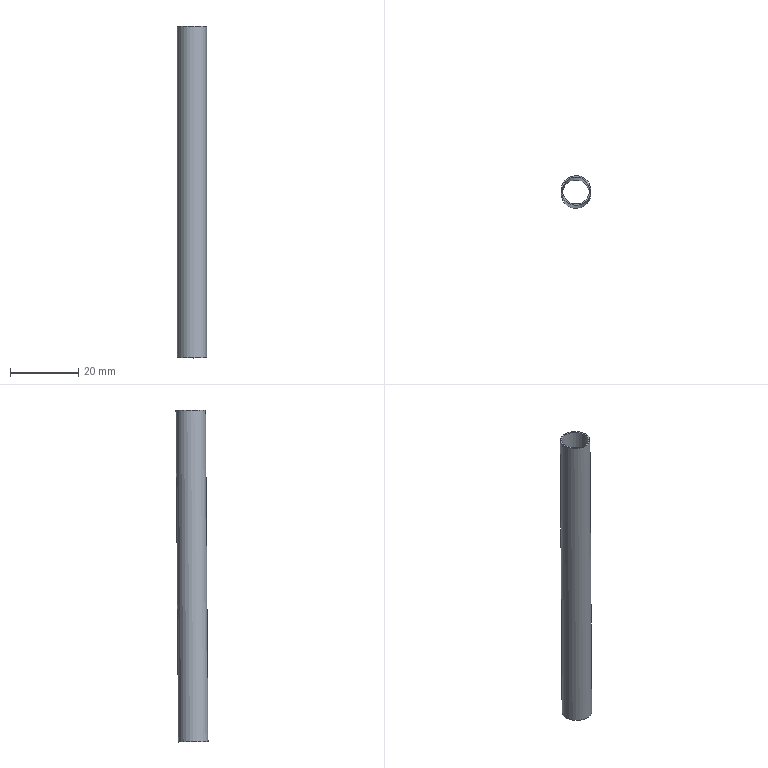Component | NX | TUBE_1 | 1 solid | 4 faces | box 8.7 x 9.44 x 97.29 mm | volume 1014 mm3 | plane 2 | cylinder 2 | commonest cylinder face diameters 8.7 x1 7.9 x1
STEP:
#1=CARTESIAN_POINT('',(0.,0.,0.));
#2=DIRECTION('',(0.,0.,1.));
#3=DIRECTION('',(1.,0.,0.));
#4=AXIS2_PLACEMENT_3D('',#1,#2,#3);
#5=CARTESIAN_POINT('',(51.171,-45.272,126.869));
#6=VERTEX_POINT('',#5);
#7=CARTESIAN_POINT('',(47.221,-45.312,126.87));
#8=DIRECTION('',(-0.0000015,-0.007573,-1.));
#9=DIRECTION('',(0.9999,0.01011,-0.00007807));
#10=AXIS2_PLACEMENT_3D('',#7,#8,#9);
#11=CIRCLE('',#10,3.95);
#12=CARTESIAN_POINT('',(47.221,-45.312,126.87));
#13=DIRECTION('',(0.0000015,0.007573,1.));
#14=DIRECTION('',(0.9999,0.01011,-0.00007807));
#15=AXIS2_PLACEMENT_3D('',#12,#13,#14);
#16=PLANE('',#15);
#17=CARTESIAN_POINT('',(3.95,0.));
#18=CARTESIAN_POINT('',(3.95,-6.842));
#19=CARTESIAN_POINT('',(-1.975,-3.421));
#20=CARTESIAN_POINT('',(-7.9,-0.));
#21=CARTESIAN_POINT('',(-1.975,3.421));
#22=CARTESIAN_POINT('',(3.95,6.842));
#23=CARTESIAN_POINT('',(3.95,0.));
#24=(BOUNDED_CURVE()B_SPLINE_CURVE(2,(#17,#18,#19,#20,#21,#22,#23),.UNSPECIFIED.,.T.,.F.)B_SPLINE_CURVE_WITH_KNOTS((1,2,2,2,2,1),(-2.094,0.,2.094,4.189,6.283,8.378),.UNSPECIFIED.)CURVE()GEOMETRIC_REPRESENTATION_ITEM()RATIONAL_B_SPLINE_CURVE((1.,0.5,1.,0.5,1.,0.5,1.))REPRESENTATION_ITEM(''));
#25=(GEOMETRIC_REPRESENTATION_CONTEXT(2)PARAMETRIC_REPRESENTATION_CONTEXT()REPRESENTATION_CONTEXT('',''));
#26=DEFINITIONAL_REPRESENTATION('',(#24),#25);
#27=PCURVE('',#16,#26);
#28=CARTESIAN_POINT('',(47.221,-46.048,29.642));
#29=DIRECTION('',(0.0000015,0.007573,1.));
#30=DIRECTION('',(0.9999,0.01011,-0.00007807));
#31=AXIS2_PLACEMENT_3D('',#28,#29,#30);
#32=CYLINDRICAL_SURFACE('',#31,3.95);
#33=CARTESIAN_POINT('',(6.283,97.23));
#34=DIRECTION('',(-1.,0.));
#35=VECTOR('',#34,1.);
#36=LINE('',#33,#35);
#37=(GEOMETRIC_REPRESENTATION_CONTEXT(2)PARAMETRIC_REPRESENTATION_CONTEXT()REPRESENTATION_CONTEXT('',''));
#38=DEFINITIONAL_REPRESENTATION('',(#36),#37);
#39=PCURVE('',#32,#38);
#40=SURFACE_CURVE('',#11,(#27,#39),.PCURVE_S1.);
#41=EDGE_CURVE('',#6,#6,#40,.T.);
#42=ORIENTED_EDGE('',*,*,#41,.T.);
#43=EDGE_LOOP('',(#42));
#44=FACE_BOUND('',#43,.T.);
#45=CARTESIAN_POINT('',(51.571,-45.268,126.869));
#46=VERTEX_POINT('',#45);
#47=CARTESIAN_POINT('',(47.221,-45.312,126.87));
#48=DIRECTION('',(-0.0000015,-0.007573,-1.));
#49=DIRECTION('',(0.9999,0.01011,-0.00007807));
#50=AXIS2_PLACEMENT_3D('',#47,#48,#49);
#51=CIRCLE('',#50,4.35);
#52=CARTESIAN_POINT('',(4.35,0.));
#53=CARTESIAN_POINT('',(4.35,-7.534));
#54=CARTESIAN_POINT('',(-2.175,-3.767));
#55=CARTESIAN_POINT('',(-8.7,-0.));
#56=CARTESIAN_POINT('',(-2.175,3.767));
#57=CARTESIAN_POINT('',(4.35,7.534));
#58=CARTESIAN_POINT('',(4.35,0.));
#59=(BOUNDED_CURVE()B_SPLINE_CURVE(2,(#52,#53,#54,#55,#56,#57,#58),.UNSPECIFIED.,.T.,.F.)B_SPLINE_CURVE_WITH_KNOTS((1,2,2,2,2,1),(-2.094,0.,2.094,4.189,6.283,8.378),.UNSPECIFIED.)CURVE()GEOMETRIC_REPRESENTATION_ITEM()RATIONAL_B_SPLINE_CURVE((1.,0.5,1.,0.5,1.,0.5,1.))REPRESENTATION_ITEM(''));
#60=(GEOMETRIC_REPRESENTATION_CONTEXT(2)PARAMETRIC_REPRESENTATION_CONTEXT()REPRESENTATION_CONTEXT('',''));
#61=DEFINITIONAL_REPRESENTATION('',(#59),#60);
#62=PCURVE('',#16,#61);
#63=CARTESIAN_POINT('',(47.221,-46.048,29.642));
#64=DIRECTION('',(0.0000015,0.007573,1.));
#65=DIRECTION('',(0.9999,0.01011,-0.00007807));
#66=AXIS2_PLACEMENT_3D('',#63,#64,#65);
#67=CYLINDRICAL_SURFACE('',#66,4.35);
#68=CARTESIAN_POINT('',(6.283,97.23));
#69=DIRECTION('',(-1.,0.));
#70=VECTOR('',#69,1.);
#71=LINE('',#68,#70);
#72=(GEOMETRIC_REPRESENTATION_CONTEXT(2)PARAMETRIC_REPRESENTATION_CONTEXT()REPRESENTATION_CONTEXT('',''));
#73=DEFINITIONAL_REPRESENTATION('',(#71),#72);
#74=PCURVE('',#67,#73);
#75=SURFACE_CURVE('',#51,(#62,#74),.PCURVE_S1.);
#76=EDGE_CURVE('',#46,#46,#75,.T.);
#77=ORIENTED_EDGE('',*,*,#76,.F.);
#78=EDGE_LOOP('',(#77));
#79=FACE_BOUND('',#78,.T.);
#80=ADVANCED_FACE('',(#44,#79),#16,.T.);
#81=CARTESIAN_POINT('',(43.271,-46.088,29.643));
#82=VERTEX_POINT('',#81);
#83=CARTESIAN_POINT('',(51.171,-46.008,29.642));
#84=VERTEX_POINT('',#83);
#85=CARTESIAN_POINT('',(47.221,-46.048,29.642));
#86=DIRECTION('',(0.0000015,0.007573,1.));
#87=DIRECTION('',(-0.9999,-0.01011,0.00007807));
#88=AXIS2_PLACEMENT_3D('',#85,#86,#87);
#89=CIRCLE('',#88,3.95);
#90=CARTESIAN_POINT('',(47.221,-46.048,29.642));
#91=DIRECTION('',(-0.0000015,-0.007573,-1.));
#92=DIRECTION('',(-0.9999,-0.01011,0.00007807));
#93=AXIS2_PLACEMENT_3D('',#90,#91,#92);
#94=PLANE('',#93);
#95=CARTESIAN_POINT('',(3.95,-0.));
#96=CARTESIAN_POINT('',(3.95,-6.842));
#97=CARTESIAN_POINT('',(-1.975,-3.421));
#98=CARTESIAN_POINT('',(-7.9,0.));
#99=CARTESIAN_POINT('',(-1.975,3.421));
#100=CARTESIAN_POINT('',(3.95,6.842));
#101=CARTESIAN_POINT('',(3.95,-0.));
#102=(BOUNDED_CURVE()B_SPLINE_CURVE(2,(#95,#96,#97,#98,#99,#100,#101),.UNSPECIFIED.,.T.,.F.)B_SPLINE_CURVE_WITH_KNOTS((1,2,2,2,2,1),(-2.094,0.,2.094,4.189,6.283,8.378),.UNSPECIFIED.)CURVE()GEOMETRIC_REPRESENTATION_ITEM()RATIONAL_B_SPLINE_CURVE((1.,0.5,1.,0.5,1.,0.5,1.))REPRESENTATION_ITEM(''));
#103=(GEOMETRIC_REPRESENTATION_CONTEXT(2)PARAMETRIC_REPRESENTATION_CONTEXT()REPRESENTATION_CONTEXT('',''));
#104=DEFINITIONAL_REPRESENTATION('',(#102),#103);
#105=PCURVE('',#94,#104);
#106=CARTESIAN_POINT('',(3.142,0.));
#107=DIRECTION('',(1.,0.));
#108=VECTOR('',#107,1.);
#109=LINE('',#106,#108);
#110=(GEOMETRIC_REPRESENTATION_CONTEXT(2)PARAMETRIC_REPRESENTATION_CONTEXT()REPRESENTATION_CONTEXT('',''));
#111=DEFINITIONAL_REPRESENTATION('',(#109),#110);
#112=PCURVE('',#32,#111);
#113=SURFACE_CURVE('',#89,(#105,#112),.PCURVE_S1.);
#114=EDGE_CURVE('',#82,#84,#113,.T.);
#115=ORIENTED_EDGE('',*,*,#114,.T.);
#116=CARTESIAN_POINT('',(47.221,-46.048,29.642));
#117=DIRECTION('',(0.0000015,0.007573,1.));
#118=DIRECTION('',(-0.9999,-0.01011,0.00007807));
#119=AXIS2_PLACEMENT_3D('',#116,#117,#118);
#120=CIRCLE('',#119,3.95);
#121=CARTESIAN_POINT('',(3.95,-0.));
#122=CARTESIAN_POINT('',(3.95,-6.842));
#123=CARTESIAN_POINT('',(-1.975,-3.421));
#124=CARTESIAN_POINT('',(-7.9,0.));
#125=CARTESIAN_POINT('',(-1.975,3.421));
#126=CARTESIAN_POINT('',(3.95,6.842));
#127=CARTESIAN_POINT('',(3.95,-0.));
#128=(BOUNDED_CURVE()B_SPLINE_CURVE(2,(#121,#122,#123,#124,#125,#126,#127),.UNSPECIFIED.,.T.,.F.)B_SPLINE_CURVE_WITH_KNOTS((1,2,2,2,2,1),(-2.094,0.,2.094,4.189,6.283,8.378),.UNSPECIFIED.)CURVE()GEOMETRIC_REPRESENTATION_ITEM()RATIONAL_B_SPLINE_CURVE((1.,0.5,1.,0.5,1.,0.5,1.))REPRESENTATION_ITEM(''));
#129=(GEOMETRIC_REPRESENTATION_CONTEXT(2)PARAMETRIC_REPRESENTATION_CONTEXT()REPRESENTATION_CONTEXT('',''));
#130=DEFINITIONAL_REPRESENTATION('',(#128),#129);
#131=PCURVE('',#94,#130);
#132=CARTESIAN_POINT('',(-3.142,0.));
#133=DIRECTION('',(1.,0.));
#134=VECTOR('',#133,1.);
#135=LINE('',#132,#134);
#136=(GEOMETRIC_REPRESENTATION_CONTEXT(2)PARAMETRIC_REPRESENTATION_CONTEXT()REPRESENTATION_CONTEXT('',''));
#137=DEFINITIONAL_REPRESENTATION('',(#135),#136);
#138=PCURVE('',#32,#137);
#139=SURFACE_CURVE('',#120,(#131,#138),.PCURVE_S1.);
#140=EDGE_CURVE('',#84,#82,#139,.T.);
#141=ORIENTED_EDGE('',*,*,#140,.T.);
#142=EDGE_LOOP('',(#115,#141));
#143=FACE_BOUND('',#142,.T.);
#144=CARTESIAN_POINT('',(51.571,-46.004,29.642));
#145=VERTEX_POINT('',#144);
#146=CARTESIAN_POINT('',(47.221,-46.048,29.642));
#147=DIRECTION('',(0.0000015,0.007573,1.));
#148=DIRECTION('',(0.9999,0.01011,-0.00007807));
#149=AXIS2_PLACEMENT_3D('',#146,#147,#148);
#150=CIRCLE('',#149,4.35);
#151=CARTESIAN_POINT('',(-4.35,0.));
#152=CARTESIAN_POINT('',(-4.35,7.534));
#153=CARTESIAN_POINT('',(2.175,3.767));
#154=CARTESIAN_POINT('',(8.7,-0.));
#155=CARTESIAN_POINT('',(2.175,-3.767));
#156=CARTESIAN_POINT('',(-4.35,-7.534));
#157=CARTESIAN_POINT('',(-4.35,0.));
#158=(BOUNDED_CURVE()B_SPLINE_CURVE(2,(#151,#152,#153,#154,#155,#156,#157),.UNSPECIFIED.,.T.,.F.)B_SPLINE_CURVE_WITH_KNOTS((1,2,2,2,2,1),(-2.094,0.,2.094,4.189,6.283,8.378),.UNSPECIFIED.)CURVE()GEOMETRIC_REPRESENTATION_ITEM()RATIONAL_B_SPLINE_CURVE((1.,0.5,1.,0.5,1.,0.5,1.))REPRESENTATION_ITEM(''));
#159=(GEOMETRIC_REPRESENTATION_CONTEXT(2)PARAMETRIC_REPRESENTATION_CONTEXT()REPRESENTATION_CONTEXT('',''));
#160=DEFINITIONAL_REPRESENTATION('',(#158),#159);
#161=PCURVE('',#94,#160);
#162=CARTESIAN_POINT('',(0.,0.));
#163=DIRECTION('',(1.,0.));
#164=VECTOR('',#163,1.);
#165=LINE('',#162,#164);
#166=(GEOMETRIC_REPRESENTATION_CONTEXT(2)PARAMETRIC_REPRESENTATION_CONTEXT()REPRESENTATION_CONTEXT('',''));
#167=DEFINITIONAL_REPRESENTATION('',(#165),#166);
#168=PCURVE('',#67,#167);
#169=SURFACE_CURVE('',#150,(#161,#168),.PCURVE_S1.);
#170=EDGE_CURVE('',#145,#145,#169,.T.);
#171=ORIENTED_EDGE('',*,*,#170,.F.);
#172=EDGE_LOOP('',(#171));
#173=FACE_BOUND('',#172,.T.);
#174=ADVANCED_FACE('',(#143,#173),#94,.T.);
#175=ORIENTED_EDGE('',*,*,#76,.T.);
#176=CARTESIAN_POINT('',(51.571,-46.004,29.642));
#177=CARTESIAN_POINT('',(51.571,-45.268,126.869));
#178=B_SPLINE_CURVE_WITH_KNOTS('',1,(#176,#177),.UNSPECIFIED.,.F.,.F.,(2,2),(0.,97.23),.PIECEWISE_BEZIER_KNOTS.);
#179=CARTESIAN_POINT('',(0.,0.));
#180=DIRECTION('',(0.,1.));
#181=VECTOR('',#180,1.);
#182=LINE('',#179,#181);
#183=(GEOMETRIC_REPRESENTATION_CONTEXT(2)PARAMETRIC_REPRESENTATION_CONTEXT()REPRESENTATION_CONTEXT('',''));
#184=DEFINITIONAL_REPRESENTATION('',(#182),#183);
#185=PCURVE('',#67,#184);
#186=CARTESIAN_POINT('',(6.283,0.));
#187=DIRECTION('',(0.,1.));
#188=VECTOR('',#187,1.);
#189=LINE('',#186,#188);
#190=(GEOMETRIC_REPRESENTATION_CONTEXT(2)PARAMETRIC_REPRESENTATION_CONTEXT()REPRESENTATION_CONTEXT('',''));
#191=DEFINITIONAL_REPRESENTATION('',(#189),#190);
#192=PCURVE('',#67,#191);
#193=SEAM_CURVE('',#178,(#185,#192),.PCURVE_S1.);
#194=EDGE_CURVE('',#145,#46,#193,.T.);
#195=ORIENTED_EDGE('',*,*,#194,.F.);
#196=ORIENTED_EDGE('',*,*,#170,.T.);
#197=ORIENTED_EDGE('',*,*,#194,.T.);
#198=EDGE_LOOP('',(#175,#195,#196,#197));
#199=FACE_BOUND('',#198,.T.);
#200=ADVANCED_FACE('',(#199),#67,.T.);
#201=ORIENTED_EDGE('',*,*,#41,.T.);
#202=CARTESIAN_POINT('',(51.171,-46.008,29.642));
#203=CARTESIAN_POINT('',(51.171,-45.272,126.869));
#204=B_SPLINE_CURVE_WITH_KNOTS('',1,(#202,#203),.UNSPECIFIED.,.F.,.F.,(2,2),(0.,97.23),.PIECEWISE_BEZIER_KNOTS.);
#205=CARTESIAN_POINT('',(0.,0.));
#206=DIRECTION('',(0.,1.));
#207=VECTOR('',#206,1.);
#208=LINE('',#205,#207);
#209=(GEOMETRIC_REPRESENTATION_CONTEXT(2)PARAMETRIC_REPRESENTATION_CONTEXT()REPRESENTATION_CONTEXT('',''));
#210=DEFINITIONAL_REPRESENTATION('',(#208),#209);
#211=PCURVE('',#32,#210);
#212=CARTESIAN_POINT('',(6.283,0.));
#213=DIRECTION('',(0.,1.));
#214=VECTOR('',#213,1.);
#215=LINE('',#212,#214);
#216=(GEOMETRIC_REPRESENTATION_CONTEXT(2)PARAMETRIC_REPRESENTATION_CONTEXT()REPRESENTATION_CONTEXT('',''));
#217=DEFINITIONAL_REPRESENTATION('',(#215),#216);
#218=PCURVE('',#32,#217);
#219=SEAM_CURVE('',#204,(#211,#218),.PCURVE_S1.);
#220=EDGE_CURVE('',#84,#6,#219,.T.);
#221=ORIENTED_EDGE('',*,*,#220,.F.);
#222=ORIENTED_EDGE('',*,*,#140,.T.);
#223=ORIENTED_EDGE('',*,*,#114,.T.);
#224=ORIENTED_EDGE('',*,*,#220,.T.);
#225=EDGE_LOOP('',(#201,#221,#222,#223,#224));
#226=FACE_BOUND('',#225,.F.);
#227=ADVANCED_FACE('',(#226),#32,.F.);
#228=CLOSED_SHELL('',(#80,#174,#200,#227));
#229=MANIFOLD_SOLID_BREP('',#228);
#230=(LENGTH_UNIT()NAMED_UNIT(*)SI_UNIT(.MILLI.,.METRE.));
#231=UNCERTAINTY_MEASURE_WITH_UNIT(LENGTH_MEASURE(0.000005),#230,'','');
#232=(NAMED_UNIT(*)PLANE_ANGLE_UNIT()SI_UNIT($,.RADIAN.));
#233=(NAMED_UNIT(*)SI_UNIT($,.STERADIAN.)SOLID_ANGLE_UNIT());
#234=(GEOMETRIC_REPRESENTATION_CONTEXT(3)GLOBAL_UNCERTAINTY_ASSIGNED_CONTEXT((#231))GLOBAL_UNIT_ASSIGNED_CONTEXT((#230,#232,#233))REPRESENTATION_CONTEXT('',''));
#235=ADVANCED_BREP_SHAPE_REPRESENTATION('',(#4,#229),#234);